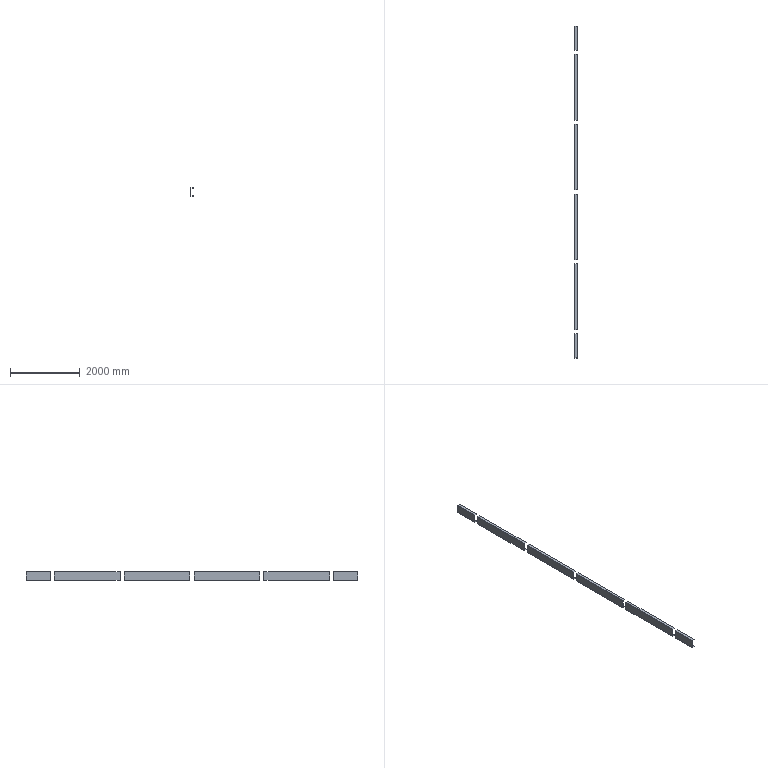Component | NX | CHUNSHUIJINCAO_5_2 | 6 solids | 60 faces | volume 35230140 mm3 | plane 60